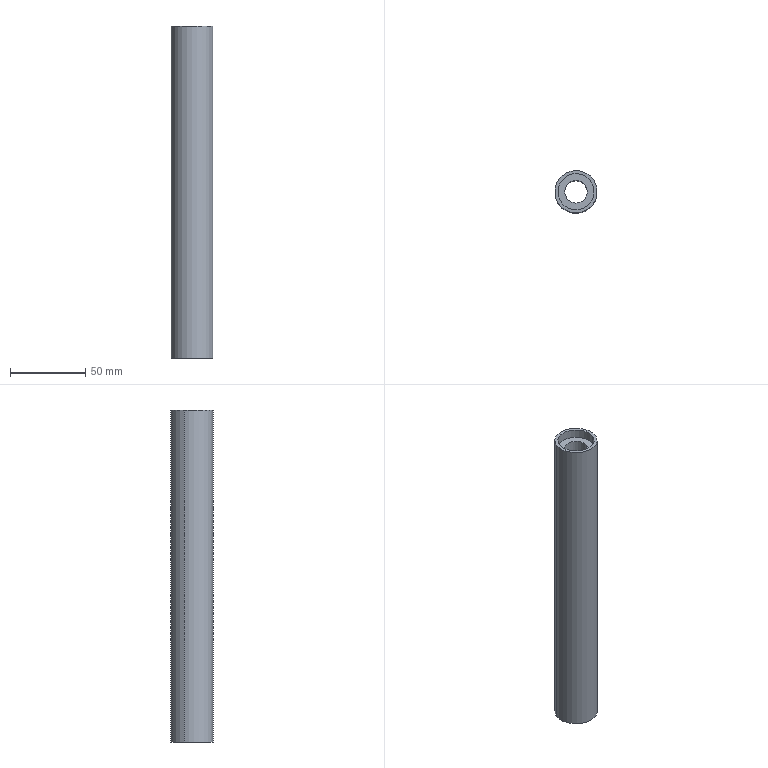Component | SolidWorks | JYTBJ-HeaderRollerBody-1_JYTBJ-HeaderRoller-1 | 1 solid | 12 faces | box 28 x 28 x 220 mm | volume 93280 mm3 | cylinder 8 | plane 4 | commonest cylinder face diameters 24 x4 28 x2 15 x2
build123d program:
from build123d import *

# Parameters (mm, degrees)
SKETCH1_R           = 14
SKETCH1_R_2         = 7.5
BOSS_EXTRUDE1_DEPTH = 110
SKETCH2_R           = 12
CUT_EXTRUDE1_DEPTH  = 6


with BuildPart() as part:
    # Sketch1 → Boss-Extrude1 (new, symmetric)
    with BuildSketch(Plane.XY):
        Circle(SKETCH1_R)
        Circle(SKETCH1_R_2, mode=Mode.SUBTRACT)
    extrude(amount=BOSS_EXTRUDE1_DEPTH, both=True)

    # Sketch2 → Cut-Extrude1 (cut)
    with BuildSketch(Plane.XY.offset(110)):
        Circle(SKETCH2_R)
    cut_extrude1 = extrude(amount=-CUT_EXTRUDE1_DEPTH, mode=Mode.SUBTRACT)

    # Mirror1: Cut-Extrude1 across plane
    add(cut_extrude1.mirror(Plane.XY), mode=Mode.SUBTRACT)


solid = part.part

# Placed as in the assembly
solid = solid.moved(Location((-199.694, 181.012, 161), (0, 0, 0)))
STEP:
#1=CARTESIAN_POINT('',(-7.421,6.956,2.244));
#2=VERTEX_POINT('',#1);
#3=CARTESIAN_POINT('',(-8.303,7.297,2.244));
#4=VERTEX_POINT('',#3);
#5=CARTESIAN_POINT('',(-7.862,7.126,2.244));
#6=DIRECTION('',(-0.,0.,1.));
#7=DIRECTION('',(-0.9328,0.3604,0.));
#8=AXIS2_PLACEMENT_3D('',#5,#6,#7);
#9=CIRCLE('',#8,0.4724);
#10=EDGE_CURVE('',#2,#4,#9,.T.);
#11=ORIENTED_EDGE('',*,*,#10,.T.);
#12=CARTESIAN_POINT('',(-8.303,7.297,2.008));
#13=VERTEX_POINT('',#12);
#14=CARTESIAN_POINT('',(-8.303,7.297,2.244));
#15=DIRECTION('',(0.,-0.,-1.));
#16=VECTOR('',#15,39.37);
#17=LINE('',#14,#16);
#18=EDGE_CURVE('',#4,#13,#17,.T.);
#19=ORIENTED_EDGE('',*,*,#18,.T.);
#20=CARTESIAN_POINT('',(-7.421,6.956,2.008));
#21=VERTEX_POINT('',#20);
#22=CARTESIAN_POINT('',(-7.862,7.126,2.008));
#23=DIRECTION('',(-0.,0.,1.));
#24=DIRECTION('',(-0.9328,0.3604,0.));
#25=AXIS2_PLACEMENT_3D('',#22,#23,#24);
#26=CIRCLE('',#25,0.4724);
#27=EDGE_CURVE('',#21,#13,#26,.T.);
#28=ORIENTED_EDGE('',*,*,#27,.F.);
#29=CARTESIAN_POINT('',(-7.421,6.956,2.244));
#30=DIRECTION('',(0.,-0.,-1.));
#31=VECTOR('',#30,39.37);
#32=LINE('',#29,#31);
#33=EDGE_CURVE('',#2,#21,#32,.T.);
#34=ORIENTED_EDGE('',*,*,#33,.F.);
#35=EDGE_LOOP('',(#11,#19,#28,#34));
#36=FACE_OUTER_BOUND('',#35,.T.);
#37=CARTESIAN_POINT('',(-7.862,7.126,2.244));
#38=DIRECTION('',(0.,-0.,-1.));
#39=DIRECTION('',(0.9328,-0.3604,0.));
#40=AXIS2_PLACEMENT_3D('',#37,#38,#39);
#41=CYLINDRICAL_SURFACE('',#40,0.4724);
#42=ADVANCED_FACE('',(#36),#41,.F.);
#43=CARTESIAN_POINT('',(-7.421,6.956,10.433));
#44=VERTEX_POINT('',#43);
#45=CARTESIAN_POINT('',(-8.303,7.297,10.433));
#46=VERTEX_POINT('',#45);
#47=CARTESIAN_POINT('',(-7.862,7.126,10.433));
#48=DIRECTION('',(-0.,0.,1.));
#49=DIRECTION('',(-0.9328,0.3604,0.));
#50=AXIS2_PLACEMENT_3D('',#47,#48,#49);
#51=CIRCLE('',#50,0.4724);
#52=EDGE_CURVE('',#44,#46,#51,.T.);
#53=ORIENTED_EDGE('',*,*,#52,.F.);
#54=CARTESIAN_POINT('',(-7.421,6.956,10.669));
#55=VERTEX_POINT('',#54);
#56=CARTESIAN_POINT('',(-7.421,6.956,10.433));
#57=DIRECTION('',(-0.,0.,1.));
#58=VECTOR('',#57,39.37);
#59=LINE('',#56,#58);
#60=EDGE_CURVE('',#44,#55,#59,.T.);
#61=ORIENTED_EDGE('',*,*,#60,.T.);
#62=CARTESIAN_POINT('',(-8.303,7.297,10.669));
#63=VERTEX_POINT('',#62);
#64=CARTESIAN_POINT('',(-7.862,7.126,10.669));
#65=DIRECTION('',(-0.,0.,1.));
#66=DIRECTION('',(-0.9328,0.3604,0.));
#67=AXIS2_PLACEMENT_3D('',#64,#65,#66);
#68=CIRCLE('',#67,0.4724);
#69=EDGE_CURVE('',#55,#63,#68,.T.);
#70=ORIENTED_EDGE('',*,*,#69,.T.);
#71=CARTESIAN_POINT('',(-8.303,7.297,10.433));
#72=DIRECTION('',(-0.,0.,1.));
#73=VECTOR('',#72,39.37);
#74=LINE('',#71,#73);
#75=EDGE_CURVE('',#46,#63,#74,.T.);
#76=ORIENTED_EDGE('',*,*,#75,.F.);
#77=EDGE_LOOP('',(#53,#61,#70,#76));
#78=FACE_OUTER_BOUND('',#77,.T.);
#79=CARTESIAN_POINT('',(-7.862,7.126,10.433));
#80=DIRECTION('',(-0.,0.,1.));
#81=DIRECTION('',(-0.9328,0.3604,0.));
#82=AXIS2_PLACEMENT_3D('',#79,#80,#81);
#83=CYLINDRICAL_SURFACE('',#82,0.4724);
#84=ADVANCED_FACE('',(#78),#83,.F.);
#85=CARTESIAN_POINT('',(-8.376,7.325,10.669));
#86=VERTEX_POINT('',#85);
#87=CARTESIAN_POINT('',(-7.348,6.928,10.669));
#88=VERTEX_POINT('',#87);
#89=CARTESIAN_POINT('',(-7.862,7.126,10.669));
#90=DIRECTION('',(-0.,0.,1.));
#91=DIRECTION('',(-0.9328,0.3604,0.));
#92=AXIS2_PLACEMENT_3D('',#89,#90,#91);
#93=CIRCLE('',#92,0.5512);
#94=EDGE_CURVE('',#86,#88,#93,.T.);
#95=ORIENTED_EDGE('',*,*,#94,.F.);
#96=CARTESIAN_POINT('',(-8.376,7.325,2.008));
#97=VERTEX_POINT('',#96);
#98=CARTESIAN_POINT('',(-8.376,7.325,10.669));
#99=DIRECTION('',(0.,-0.,-1.));
#100=VECTOR('',#99,39.37);
#101=LINE('',#98,#100);
#102=EDGE_CURVE('',#86,#97,#101,.T.);
#103=ORIENTED_EDGE('',*,*,#102,.T.);
#104=CARTESIAN_POINT('',(-7.348,6.928,2.008));
#105=VERTEX_POINT('',#104);
#106=CARTESIAN_POINT('',(-7.862,7.126,2.008));
#107=DIRECTION('',(-0.,0.,1.));
#108=DIRECTION('',(-0.9328,0.3604,0.));
#109=AXIS2_PLACEMENT_3D('',#106,#107,#108);
#110=CIRCLE('',#109,0.5512);
#111=EDGE_CURVE('',#97,#105,#110,.T.);
#112=ORIENTED_EDGE('',*,*,#111,.T.);
#113=CARTESIAN_POINT('',(-7.348,6.928,10.669));
#114=DIRECTION('',(0.,-0.,-1.));
#115=VECTOR('',#114,39.37);
#116=LINE('',#113,#115);
#117=EDGE_CURVE('',#88,#105,#116,.T.);
#118=ORIENTED_EDGE('',*,*,#117,.F.);
#119=EDGE_LOOP('',(#95,#103,#112,#118));
#120=FACE_OUTER_BOUND('',#119,.T.);
#121=CARTESIAN_POINT('',(-7.862,7.126,10.669));
#122=DIRECTION('',(0.,-0.,-1.));
#123=DIRECTION('',(0.9328,-0.3604,0.));
#124=AXIS2_PLACEMENT_3D('',#121,#122,#123);
#125=CYLINDRICAL_SURFACE('',#124,0.5512);
#126=ADVANCED_FACE('',(#120),#125,.T.);
#127=CARTESIAN_POINT('',(-7.587,7.02,10.433));
#128=VERTEX_POINT('',#127);
#129=CARTESIAN_POINT('',(-8.137,7.233,10.433));
#130=VERTEX_POINT('',#129);
#131=CARTESIAN_POINT('',(-7.862,7.126,10.433));
#132=DIRECTION('',(-0.,0.,1.));
#133=DIRECTION('',(-0.9328,0.3604,0.));
#134=AXIS2_PLACEMENT_3D('',#131,#132,#133);
#135=CIRCLE('',#134,0.2953);
#136=EDGE_CURVE('',#128,#130,#135,.T.);
#137=ORIENTED_EDGE('',*,*,#136,.T.);
#138=CARTESIAN_POINT('',(-8.137,7.233,2.244));
#139=VERTEX_POINT('',#138);
#140=CARTESIAN_POINT('',(-8.137,7.233,10.669));
#141=DIRECTION('',(0.,-0.,-1.));
#142=VECTOR('',#141,39.37);
#143=LINE('',#140,#142);
#144=EDGE_CURVE('',#130,#139,#143,.T.);
#145=ORIENTED_EDGE('',*,*,#144,.T.);
#146=CARTESIAN_POINT('',(-7.587,7.02,2.244));
#147=VERTEX_POINT('',#146);
#148=CARTESIAN_POINT('',(-7.862,7.126,2.244));
#149=DIRECTION('',(0.,-0.,-1.));
#150=DIRECTION('',(0.9328,-0.3604,0.));
#151=AXIS2_PLACEMENT_3D('',#148,#149,#150);
#152=CIRCLE('',#151,0.2953);
#153=EDGE_CURVE('',#139,#147,#152,.T.);
#154=ORIENTED_EDGE('',*,*,#153,.T.);
#155=CARTESIAN_POINT('',(-7.587,7.02,10.669));
#156=DIRECTION('',(0.,-0.,-1.));
#157=VECTOR('',#156,39.37);
#158=LINE('',#155,#157);
#159=EDGE_CURVE('',#128,#147,#158,.T.);
#160=ORIENTED_EDGE('',*,*,#159,.F.);
#161=EDGE_LOOP('',(#137,#145,#154,#160));
#162=FACE_OUTER_BOUND('',#161,.T.);
#163=CARTESIAN_POINT('',(-7.862,7.126,10.669));
#164=DIRECTION('',(0.,-0.,-1.));
#165=DIRECTION('',(0.9328,-0.3604,0.));
#166=AXIS2_PLACEMENT_3D('',#163,#164,#165);
#167=CYLINDRICAL_SURFACE('',#166,0.2953);
#168=ADVANCED_FACE('',(#162),#167,.F.);
#169=ORIENTED_EDGE('',*,*,#144,.F.);
#170=CARTESIAN_POINT('',(-7.862,7.126,10.433));
#171=DIRECTION('',(-0.,0.,1.));
#172=DIRECTION('',(-0.9328,0.3604,0.));
#173=AXIS2_PLACEMENT_3D('',#170,#171,#172);
#174=CIRCLE('',#173,0.2953);
#175=EDGE_CURVE('',#130,#128,#174,.T.);
#176=ORIENTED_EDGE('',*,*,#175,.T.);
#177=ORIENTED_EDGE('',*,*,#159,.T.);
#178=CARTESIAN_POINT('',(-7.862,7.126,2.244));
#179=DIRECTION('',(0.,-0.,-1.));
#180=DIRECTION('',(0.9328,-0.3604,0.));
#181=AXIS2_PLACEMENT_3D('',#178,#179,#180);
#182=CIRCLE('',#181,0.2953);
#183=EDGE_CURVE('',#147,#139,#182,.T.);
#184=ORIENTED_EDGE('',*,*,#183,.T.);
#185=EDGE_LOOP('',(#169,#176,#177,#184));
#186=FACE_OUTER_BOUND('',#185,.T.);
#187=CARTESIAN_POINT('',(-7.862,7.126,10.669));
#188=DIRECTION('',(0.,-0.,-1.));
#189=DIRECTION('',(0.9328,-0.3604,0.));
#190=AXIS2_PLACEMENT_3D('',#187,#188,#189);
#191=CYLINDRICAL_SURFACE('',#190,0.2953);
#192=ADVANCED_FACE('',(#186),#191,.F.);
#193=CARTESIAN_POINT('',(-7.862,7.126,2.008));
#194=DIRECTION('',(-0.,0.,1.));
#195=DIRECTION('',(-0.9328,0.3604,0.));
#196=AXIS2_PLACEMENT_3D('',#193,#194,#195);
#197=CIRCLE('',#196,0.5512);
#198=EDGE_CURVE('',#105,#97,#197,.T.);
#199=ORIENTED_EDGE('',*,*,#198,.F.);
#200=ORIENTED_EDGE('',*,*,#111,.F.);
#201=EDGE_LOOP('',(#199,#200));
#202=FACE_OUTER_BOUND('',#201,.T.);
#203=ORIENTED_EDGE('',*,*,#27,.T.);
#204=CARTESIAN_POINT('',(-7.862,7.126,2.008));
#205=DIRECTION('',(-0.,0.,1.));
#206=DIRECTION('',(-0.9328,0.3604,0.));
#207=AXIS2_PLACEMENT_3D('',#204,#205,#206);
#208=CIRCLE('',#207,0.4724);
#209=EDGE_CURVE('',#13,#21,#208,.T.);
#210=ORIENTED_EDGE('',*,*,#209,.T.);
#211=EDGE_LOOP('',(#203,#210));
#212=FACE_BOUND('',#211,.T.);
#213=CARTESIAN_POINT('',(-7.862,7.126,2.008));
#214=DIRECTION('',(-0.,0.,1.));
#215=DIRECTION('',(-0.9328,0.3604,-0.));
#216=AXIS2_PLACEMENT_3D('',#213,#214,#215);
#217=PLANE('',#216);
#218=ADVANCED_FACE('',(#202,#212),#217,.F.);
#219=CARTESIAN_POINT('',(-7.862,7.126,10.669));
#220=DIRECTION('',(-0.,0.,1.));
#221=DIRECTION('',(-0.9328,0.3604,0.));
#222=AXIS2_PLACEMENT_3D('',#219,#220,#221);
#223=CIRCLE('',#222,0.4724);
#224=EDGE_CURVE('',#63,#55,#223,.T.);
#225=ORIENTED_EDGE('',*,*,#224,.F.);
#226=ORIENTED_EDGE('',*,*,#69,.F.);
#227=EDGE_LOOP('',(#225,#226));
#228=FACE_BOUND('',#227,.T.);
#229=CARTESIAN_POINT('',(-7.862,7.126,10.669));
#230=DIRECTION('',(-0.,0.,1.));
#231=DIRECTION('',(-0.9328,0.3604,0.));
#232=AXIS2_PLACEMENT_3D('',#229,#230,#231);
#233=CIRCLE('',#232,0.5512);
#234=EDGE_CURVE('',#88,#86,#233,.T.);
#235=ORIENTED_EDGE('',*,*,#234,.T.);
#236=ORIENTED_EDGE('',*,*,#94,.T.);
#237=EDGE_LOOP('',(#235,#236));
#238=FACE_OUTER_BOUND('',#237,.T.);
#239=CARTESIAN_POINT('',(-7.862,7.126,10.669));
#240=DIRECTION('',(-0.,0.,1.));
#241=DIRECTION('',(-0.9328,0.3604,-0.));
#242=AXIS2_PLACEMENT_3D('',#239,#240,#241);
#243=PLANE('',#242);
#244=ADVANCED_FACE('',(#228,#238),#243,.T.);
#245=ORIENTED_EDGE('',*,*,#102,.F.);
#246=ORIENTED_EDGE('',*,*,#234,.F.);
#247=ORIENTED_EDGE('',*,*,#117,.T.);
#248=ORIENTED_EDGE('',*,*,#198,.T.);
#249=EDGE_LOOP('',(#245,#246,#247,#248));
#250=FACE_OUTER_BOUND('',#249,.T.);
#251=CARTESIAN_POINT('',(-7.862,7.126,10.669));
#252=DIRECTION('',(0.,-0.,-1.));
#253=DIRECTION('',(0.9328,-0.3604,0.));
#254=AXIS2_PLACEMENT_3D('',#251,#252,#253);
#255=CYLINDRICAL_SURFACE('',#254,0.5512);
#256=ADVANCED_FACE('',(#250),#255,.T.);
#257=ORIENTED_EDGE('',*,*,#60,.F.);
#258=CARTESIAN_POINT('',(-7.862,7.126,10.433));
#259=DIRECTION('',(-0.,0.,1.));
#260=DIRECTION('',(-0.9328,0.3604,0.));
#261=AXIS2_PLACEMENT_3D('',#258,#259,#260);
#262=CIRCLE('',#261,0.4724);
#263=EDGE_CURVE('',#46,#44,#262,.T.);
#264=ORIENTED_EDGE('',*,*,#263,.F.);
#265=ORIENTED_EDGE('',*,*,#75,.T.);
#266=ORIENTED_EDGE('',*,*,#224,.T.);
#267=EDGE_LOOP('',(#257,#264,#265,#266));
#268=FACE_OUTER_BOUND('',#267,.T.);
#269=CARTESIAN_POINT('',(-7.862,7.126,10.433));
#270=DIRECTION('',(-0.,0.,1.));
#271=DIRECTION('',(-0.9328,0.3604,0.));
#272=AXIS2_PLACEMENT_3D('',#269,#270,#271);
#273=CYLINDRICAL_SURFACE('',#272,0.4724);
#274=ADVANCED_FACE('',(#268),#273,.F.);
#275=ORIENTED_EDGE('',*,*,#136,.F.);
#276=ORIENTED_EDGE('',*,*,#175,.F.);
#277=EDGE_LOOP('',(#275,#276));
#278=FACE_BOUND('',#277,.T.);
#279=ORIENTED_EDGE('',*,*,#263,.T.);
#280=ORIENTED_EDGE('',*,*,#52,.T.);
#281=EDGE_LOOP('',(#279,#280));
#282=FACE_OUTER_BOUND('',#281,.T.);
#283=CARTESIAN_POINT('',(-7.862,7.126,10.433));
#284=DIRECTION('',(-0.,0.,1.));
#285=DIRECTION('',(-0.9328,0.3604,-0.));
#286=AXIS2_PLACEMENT_3D('',#283,#284,#285);
#287=PLANE('',#286);
#288=ADVANCED_FACE('',(#278,#282),#287,.T.);
#289=ORIENTED_EDGE('',*,*,#18,.F.);
#290=CARTESIAN_POINT('',(-7.862,7.126,2.244));
#291=DIRECTION('',(-0.,0.,1.));
#292=DIRECTION('',(-0.9328,0.3604,0.));
#293=AXIS2_PLACEMENT_3D('',#290,#291,#292);
#294=CIRCLE('',#293,0.4724);
#295=EDGE_CURVE('',#4,#2,#294,.T.);
#296=ORIENTED_EDGE('',*,*,#295,.T.);
#297=ORIENTED_EDGE('',*,*,#33,.T.);
#298=ORIENTED_EDGE('',*,*,#209,.F.);
#299=EDGE_LOOP('',(#289,#296,#297,#298));
#300=FACE_OUTER_BOUND('',#299,.T.);
#301=CARTESIAN_POINT('',(-7.862,7.126,2.244));
#302=DIRECTION('',(0.,-0.,-1.));
#303=DIRECTION('',(0.9328,-0.3604,0.));
#304=AXIS2_PLACEMENT_3D('',#301,#302,#303);
#305=CYLINDRICAL_SURFACE('',#304,0.4724);
#306=ADVANCED_FACE('',(#300),#305,.F.);
#307=ORIENTED_EDGE('',*,*,#183,.F.);
#308=ORIENTED_EDGE('',*,*,#153,.F.);
#309=EDGE_LOOP('',(#307,#308));
#310=FACE_BOUND('',#309,.T.);
#311=ORIENTED_EDGE('',*,*,#10,.F.);
#312=ORIENTED_EDGE('',*,*,#295,.F.);
#313=EDGE_LOOP('',(#311,#312));
#314=FACE_OUTER_BOUND('',#313,.T.);
#315=CARTESIAN_POINT('',(-7.862,7.126,2.244));
#316=DIRECTION('',(0.,-0.,-1.));
#317=DIRECTION('',(-0.9328,0.3604,-0.));
#318=AXIS2_PLACEMENT_3D('',#315,#316,#317);
#319=PLANE('',#318);
#320=ADVANCED_FACE('',(#310,#314),#319,.T.);
#321=CLOSED_SHELL('',(#42,#84,#126,#168,#192,#218,#244,#256,#274,#288,#306,#320));
#322=MANIFOLD_SOLID_BREP('',#321);
#323=CARTESIAN_POINT('',(0.,0.,0.));
#324=DIRECTION('',(0.,0.,1.));
#325=DIRECTION('',(1.,0.,0.));
#326=AXIS2_PLACEMENT_3D('',#323,#324,#325);
#327=(LENGTH_UNIT()NAMED_UNIT(*)SI_UNIT($,.METRE.));
#328=LENGTH_MEASURE_WITH_UNIT(LENGTH_MEASURE(0.0254),#327);
#329=DIMENSIONAL_EXPONENTS(1.,0.,0.,0.,0.,0.,0.);
#330=(CONVERSION_BASED_UNIT('',#328)LENGTH_UNIT()NAMED_UNIT(#329));
#331=UNCERTAINTY_MEASURE_WITH_UNIT(LENGTH_MEASURE(0.00001),#330,'','');
#332=(NAMED_UNIT(*)PLANE_ANGLE_UNIT()SI_UNIT($,.RADIAN.));
#333=(NAMED_UNIT(*)SI_UNIT($,.STERADIAN.)SOLID_ANGLE_UNIT());
#334=(GEOMETRIC_REPRESENTATION_CONTEXT(3)GLOBAL_UNCERTAINTY_ASSIGNED_CONTEXT((#331))GLOBAL_UNIT_ASSIGNED_CONTEXT((#330,#332,#333))REPRESENTATION_CONTEXT('',''));
#335=ADVANCED_BREP_SHAPE_REPRESENTATION('',(#322,#326),#334);
#336=COLOUR_RGB('',0.7922,0.8196,0.9333);
#337=FILL_AREA_STYLE_COLOUR('',#336);
#338=FILL_AREA_STYLE('',(#337));
#339=SURFACE_STYLE_FILL_AREA(#338);
#340=SURFACE_SIDE_STYLE('',(#339));
#341=SURFACE_STYLE_USAGE(.BOTH.,#340);
#342=PRESENTATION_STYLE_ASSIGNMENT((#341));
#343=STYLED_ITEM('',(#342),#322);
#344=PRESENTATION_LAYER_ASSIGNMENT('','',(#343));
#345=(LENGTH_UNIT()NAMED_UNIT(*)SI_UNIT($,.METRE.));
#346=LENGTH_MEASURE_WITH_UNIT(LENGTH_MEASURE(0.0254),#345);
#347=DIMENSIONAL_EXPONENTS(1.,0.,0.,0.,0.,0.,0.);
#348=(CONVERSION_BASED_UNIT('',#346)LENGTH_UNIT()NAMED_UNIT(#347));
#349=UNCERTAINTY_MEASURE_WITH_UNIT(LENGTH_MEASURE(0.00001),#348,'','');
#350=(NAMED_UNIT(*)PLANE_ANGLE_UNIT()SI_UNIT($,.RADIAN.));
#351=(NAMED_UNIT(*)SI_UNIT($,.STERADIAN.)SOLID_ANGLE_UNIT());
#352=(GEOMETRIC_REPRESENTATION_CONTEXT(3)GLOBAL_UNCERTAINTY_ASSIGNED_CONTEXT((#349))GLOBAL_UNIT_ASSIGNED_CONTEXT((#348,#350,#351))REPRESENTATION_CONTEXT('',''));
#353=MECHANICAL_DESIGN_GEOMETRIC_PRESENTATION_REPRESENTATION('',(#343),#352);